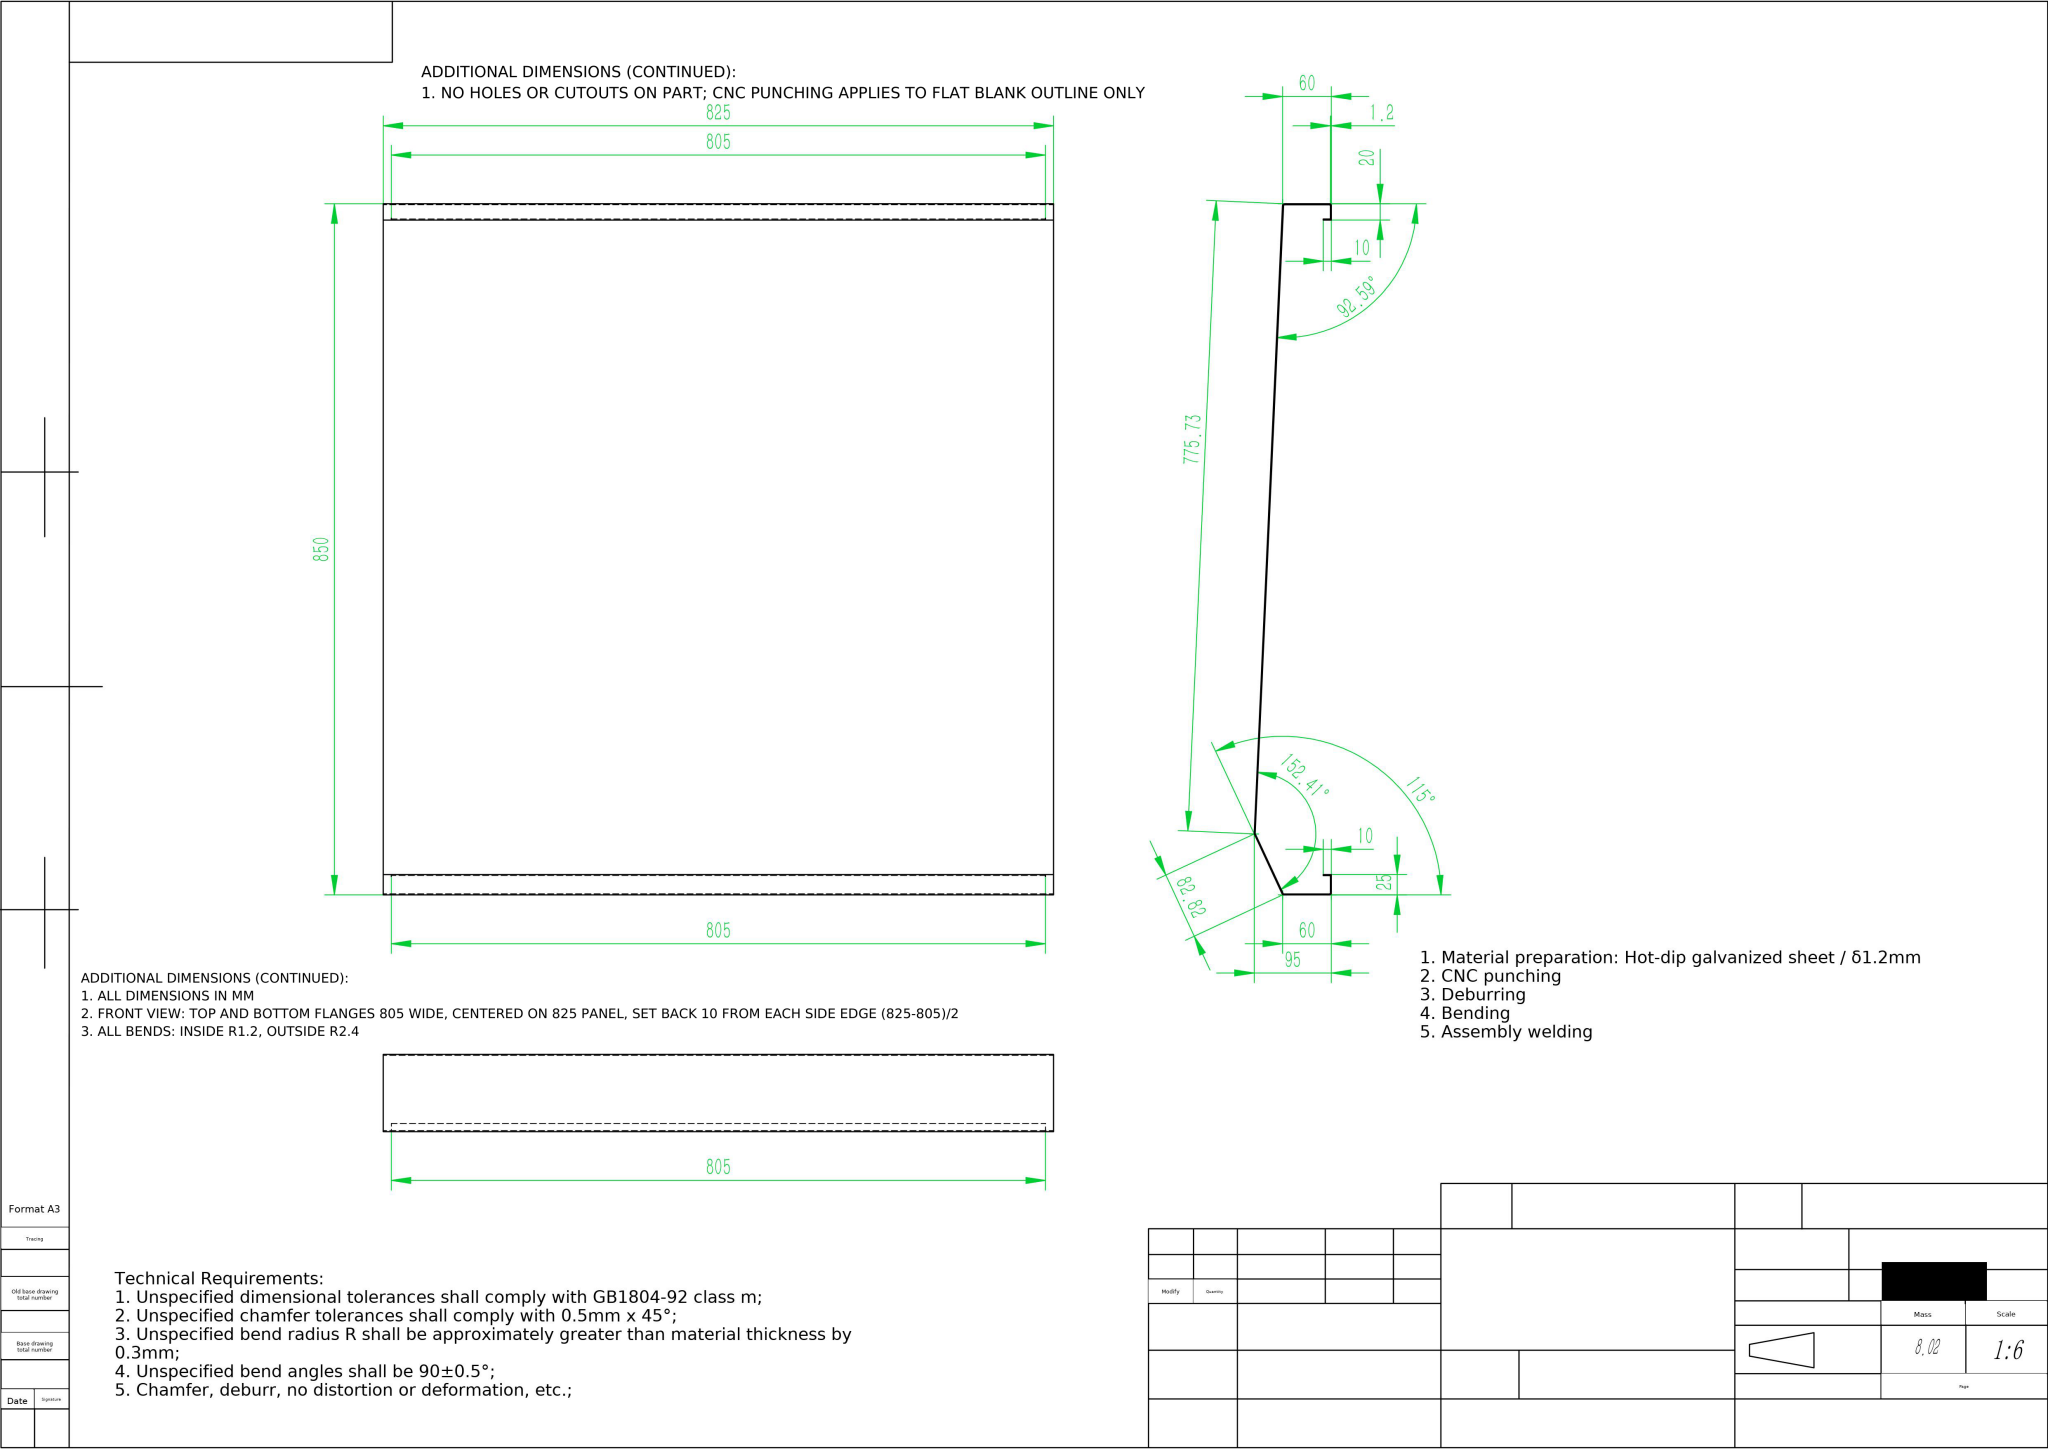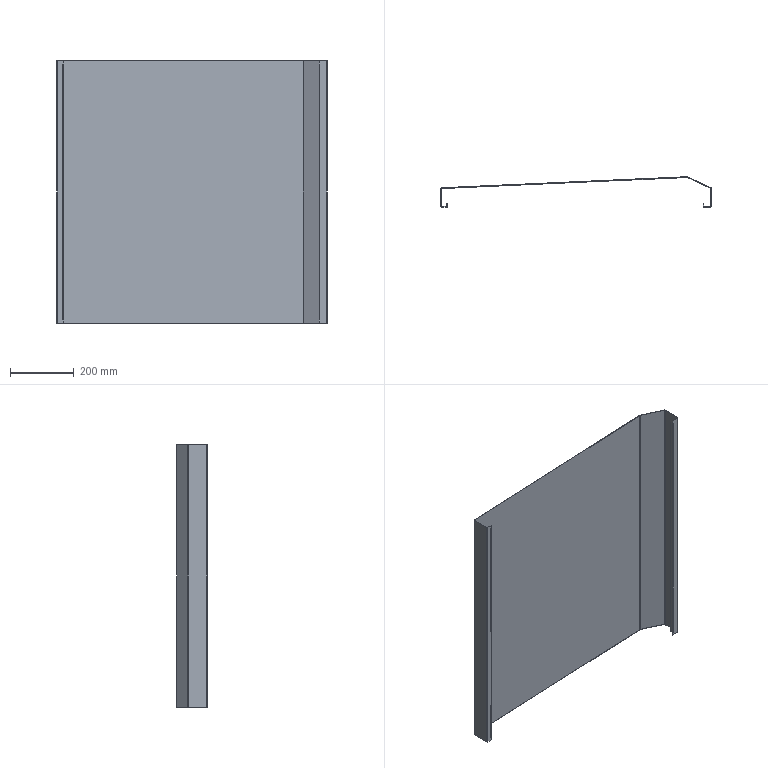Part | NX | mm | 1 solid | 70 faces | box 850 x 94.98 x 825 mm | volume 1021779 mm3 | plane 56 | cylinder 14 | commonest cylinder face diameters 2.4 x7 4.8 x7